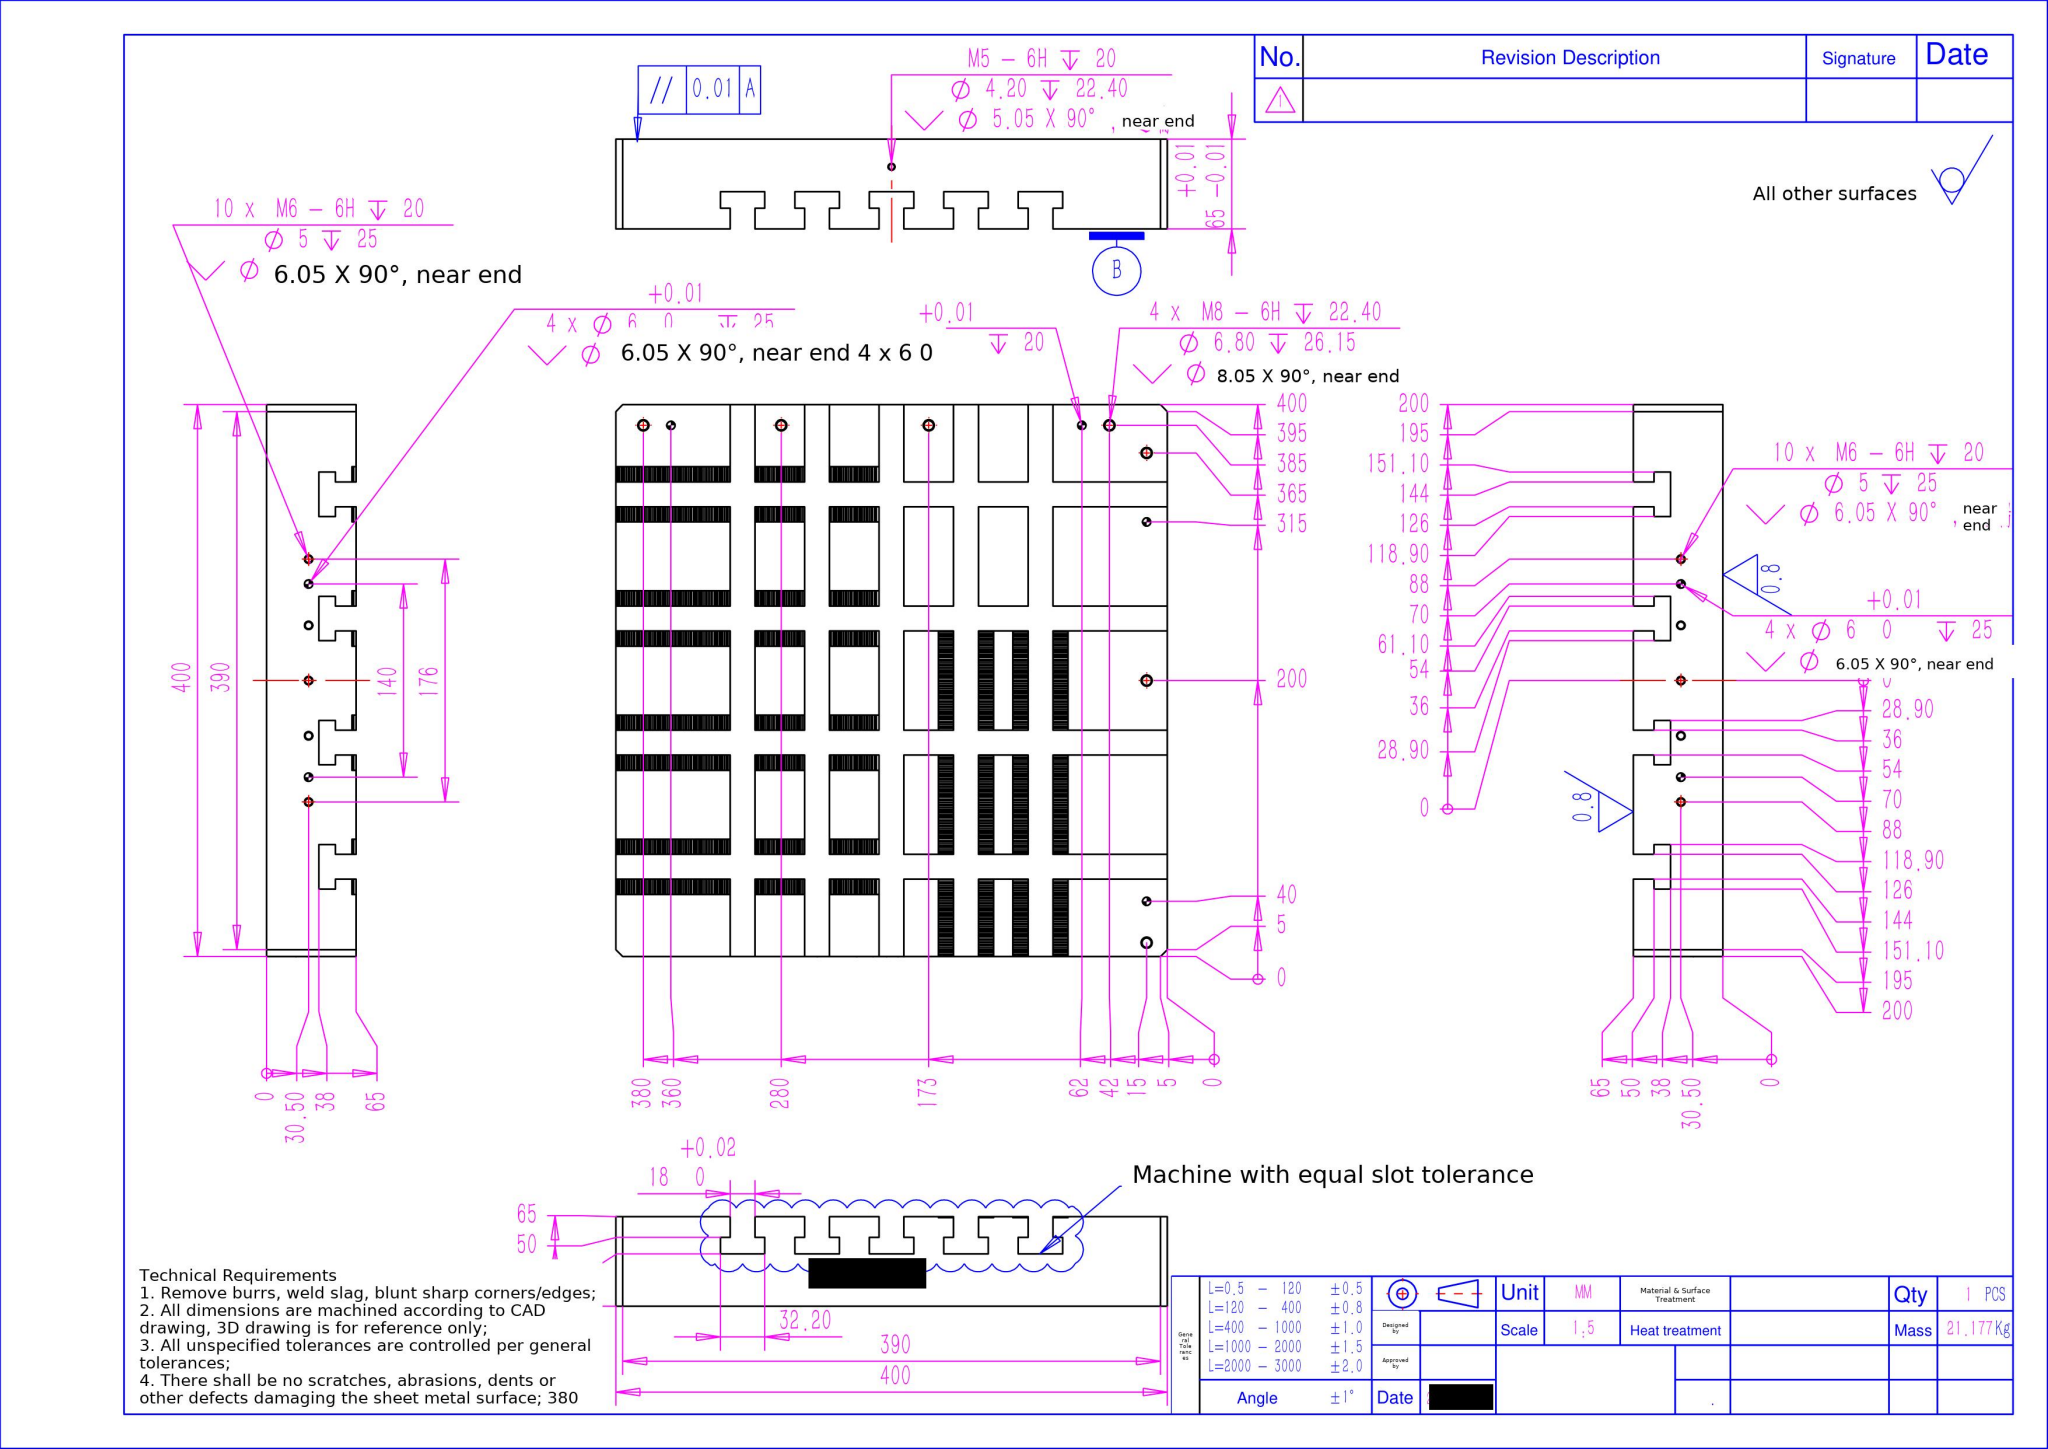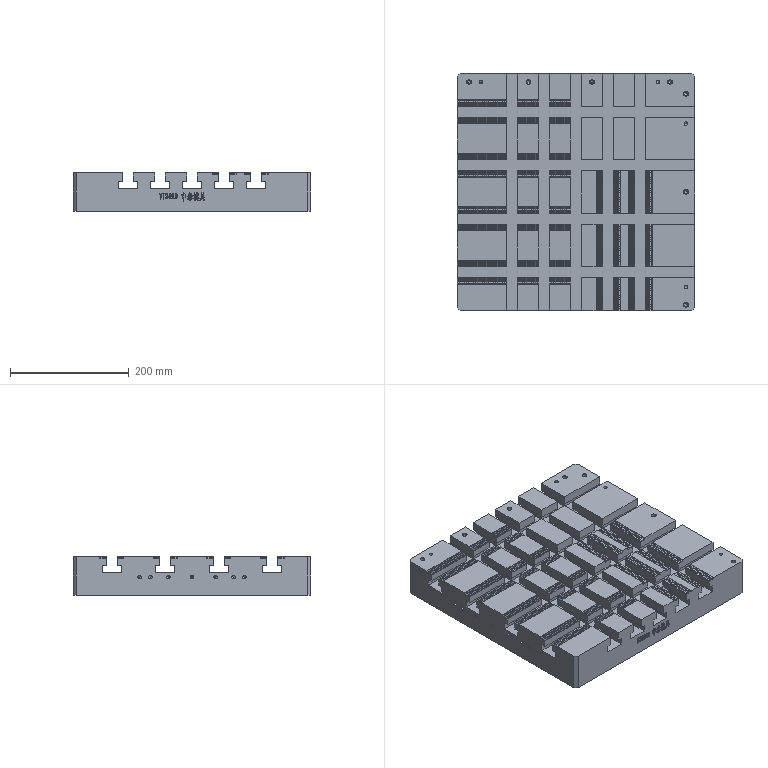Part | SolidWorks | 1 solid | 3756 faces | box 400 x 400 x 65 mm | volume 7843314 mm3 | plane 3401 | spline 165 | cone 104 | cylinder 86 | commonest cylinder face diameters 5 x20 50 x16 6 x16 6.8 x14 8.5 x8 18.02 x8 4.2 x2 200 x2